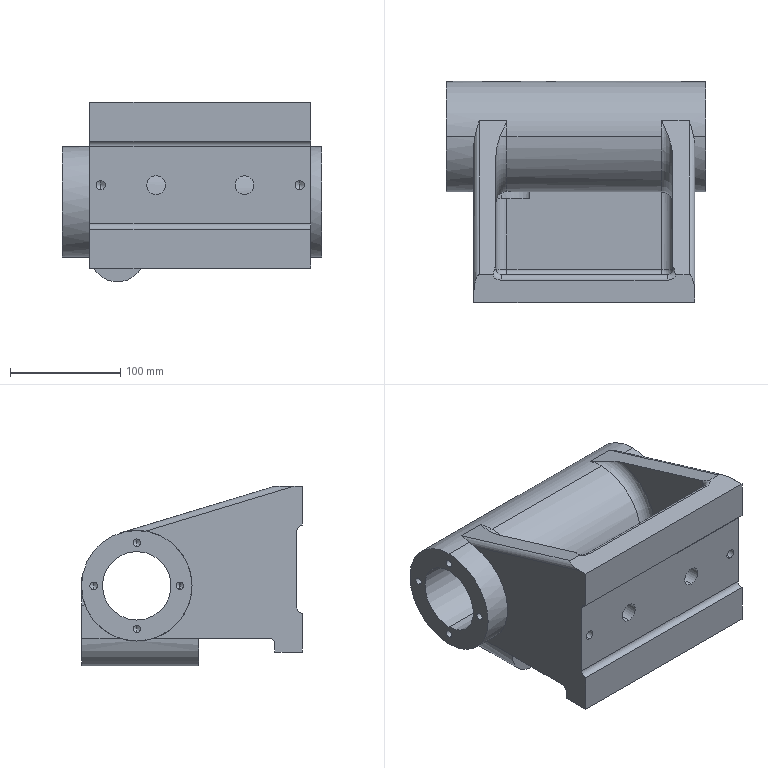Component | SolidWorks | TailstockBody-1 | 1 solid | 108 faces | volume 2563814 mm3 | cylinder 54 | plane 24 | cone 22 | torus 8 | commonest cylinder face diameters 6.8 x16 10 x9 50 x7 8.5 x6 17 x4 100 x4 20 x4 25 x2